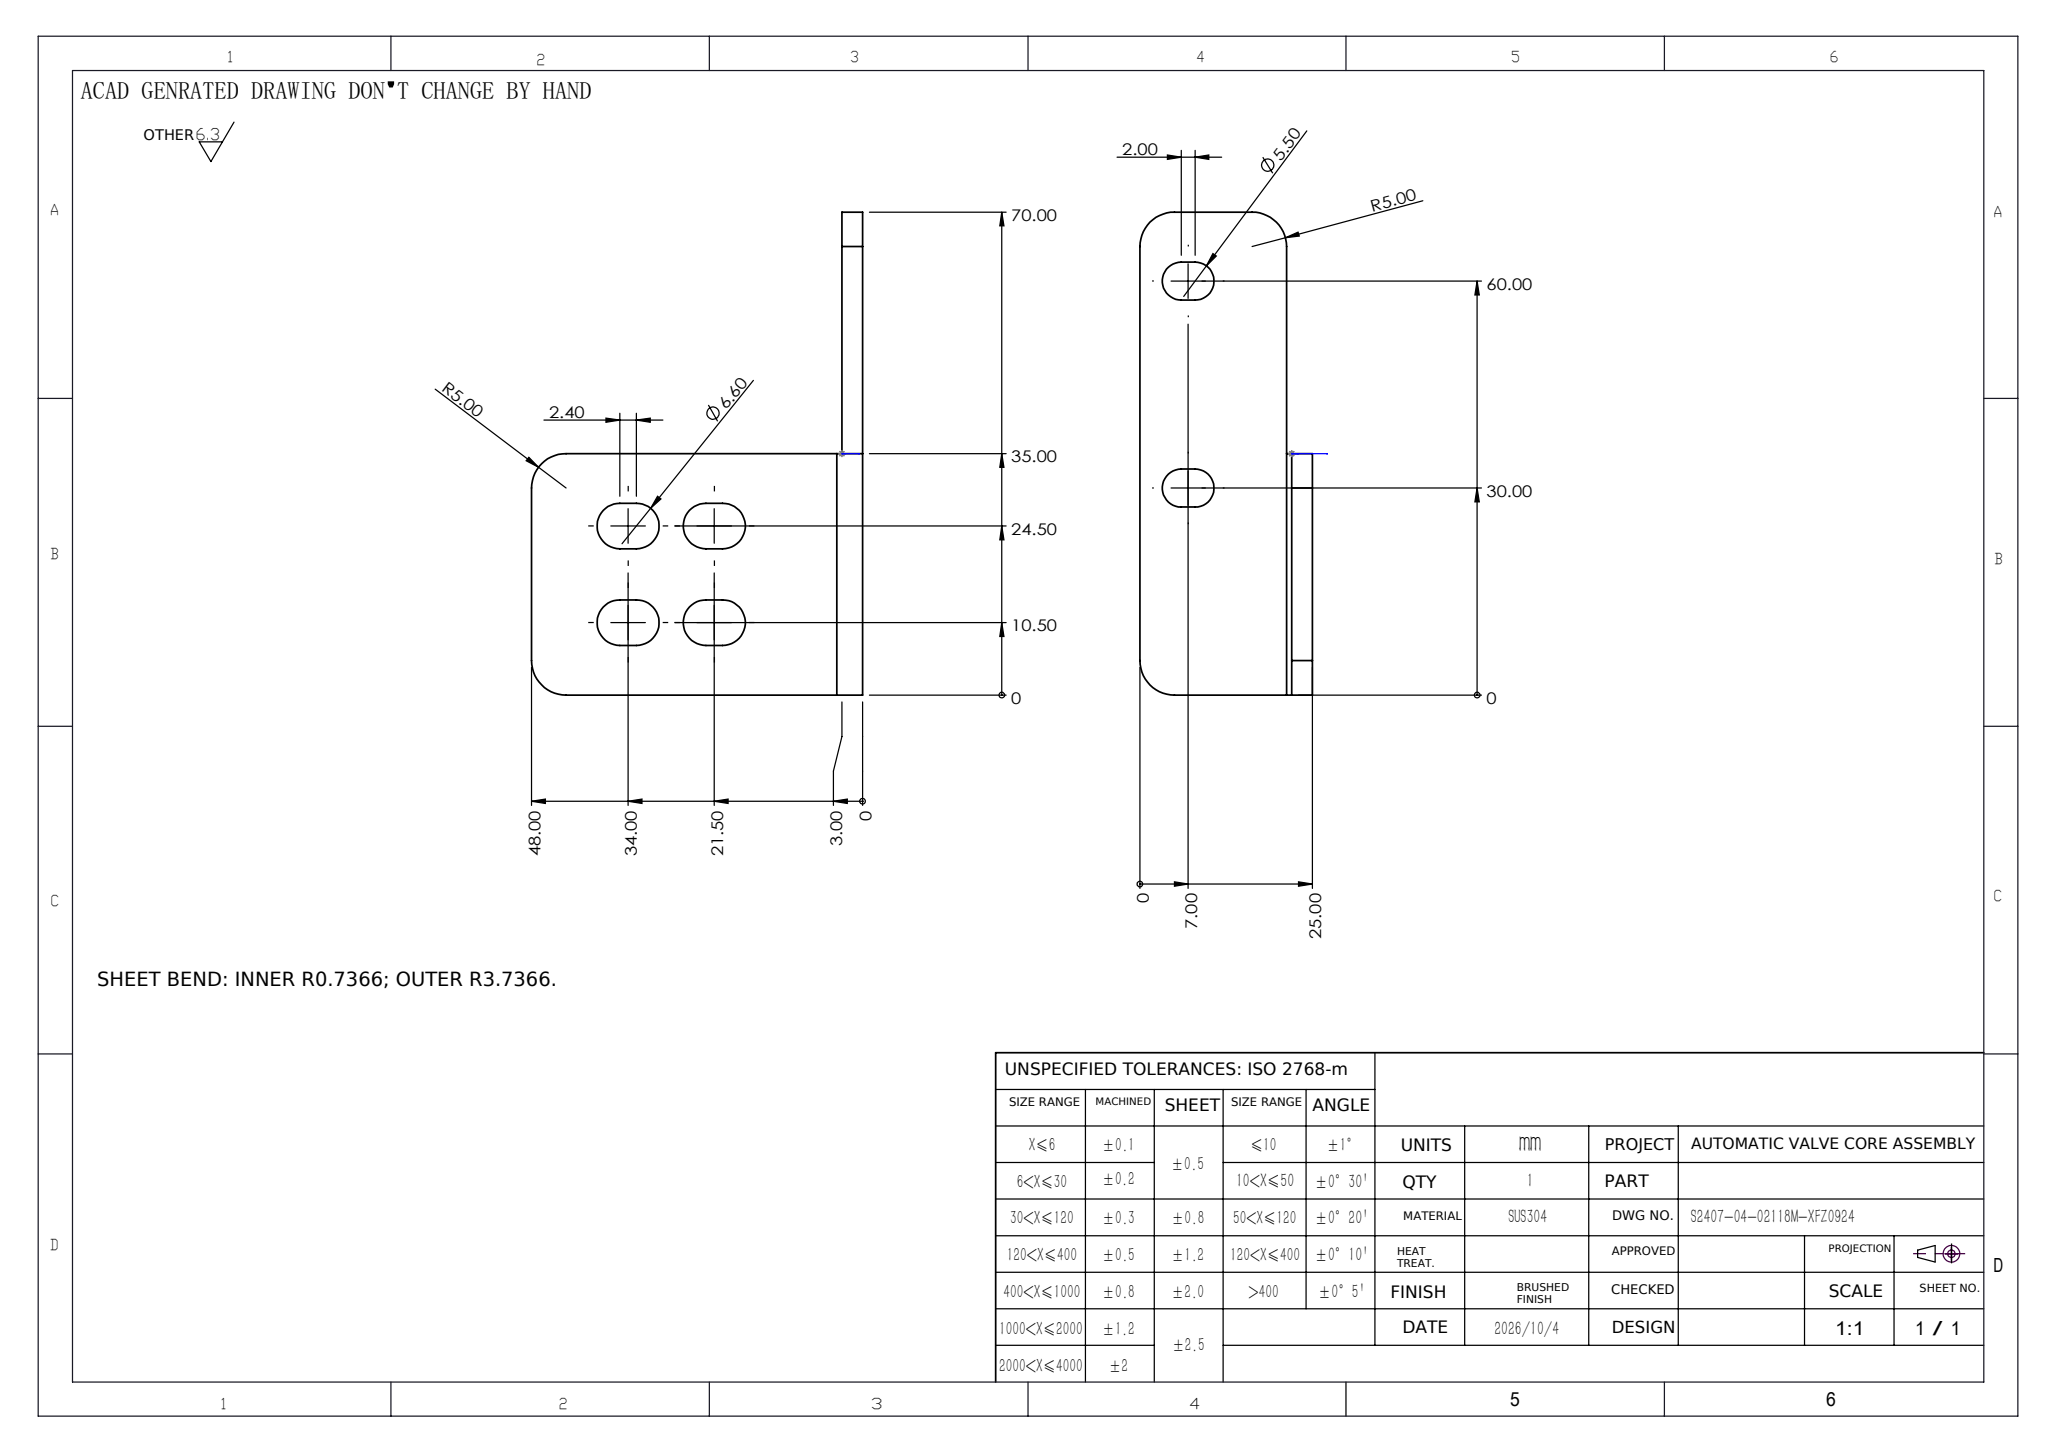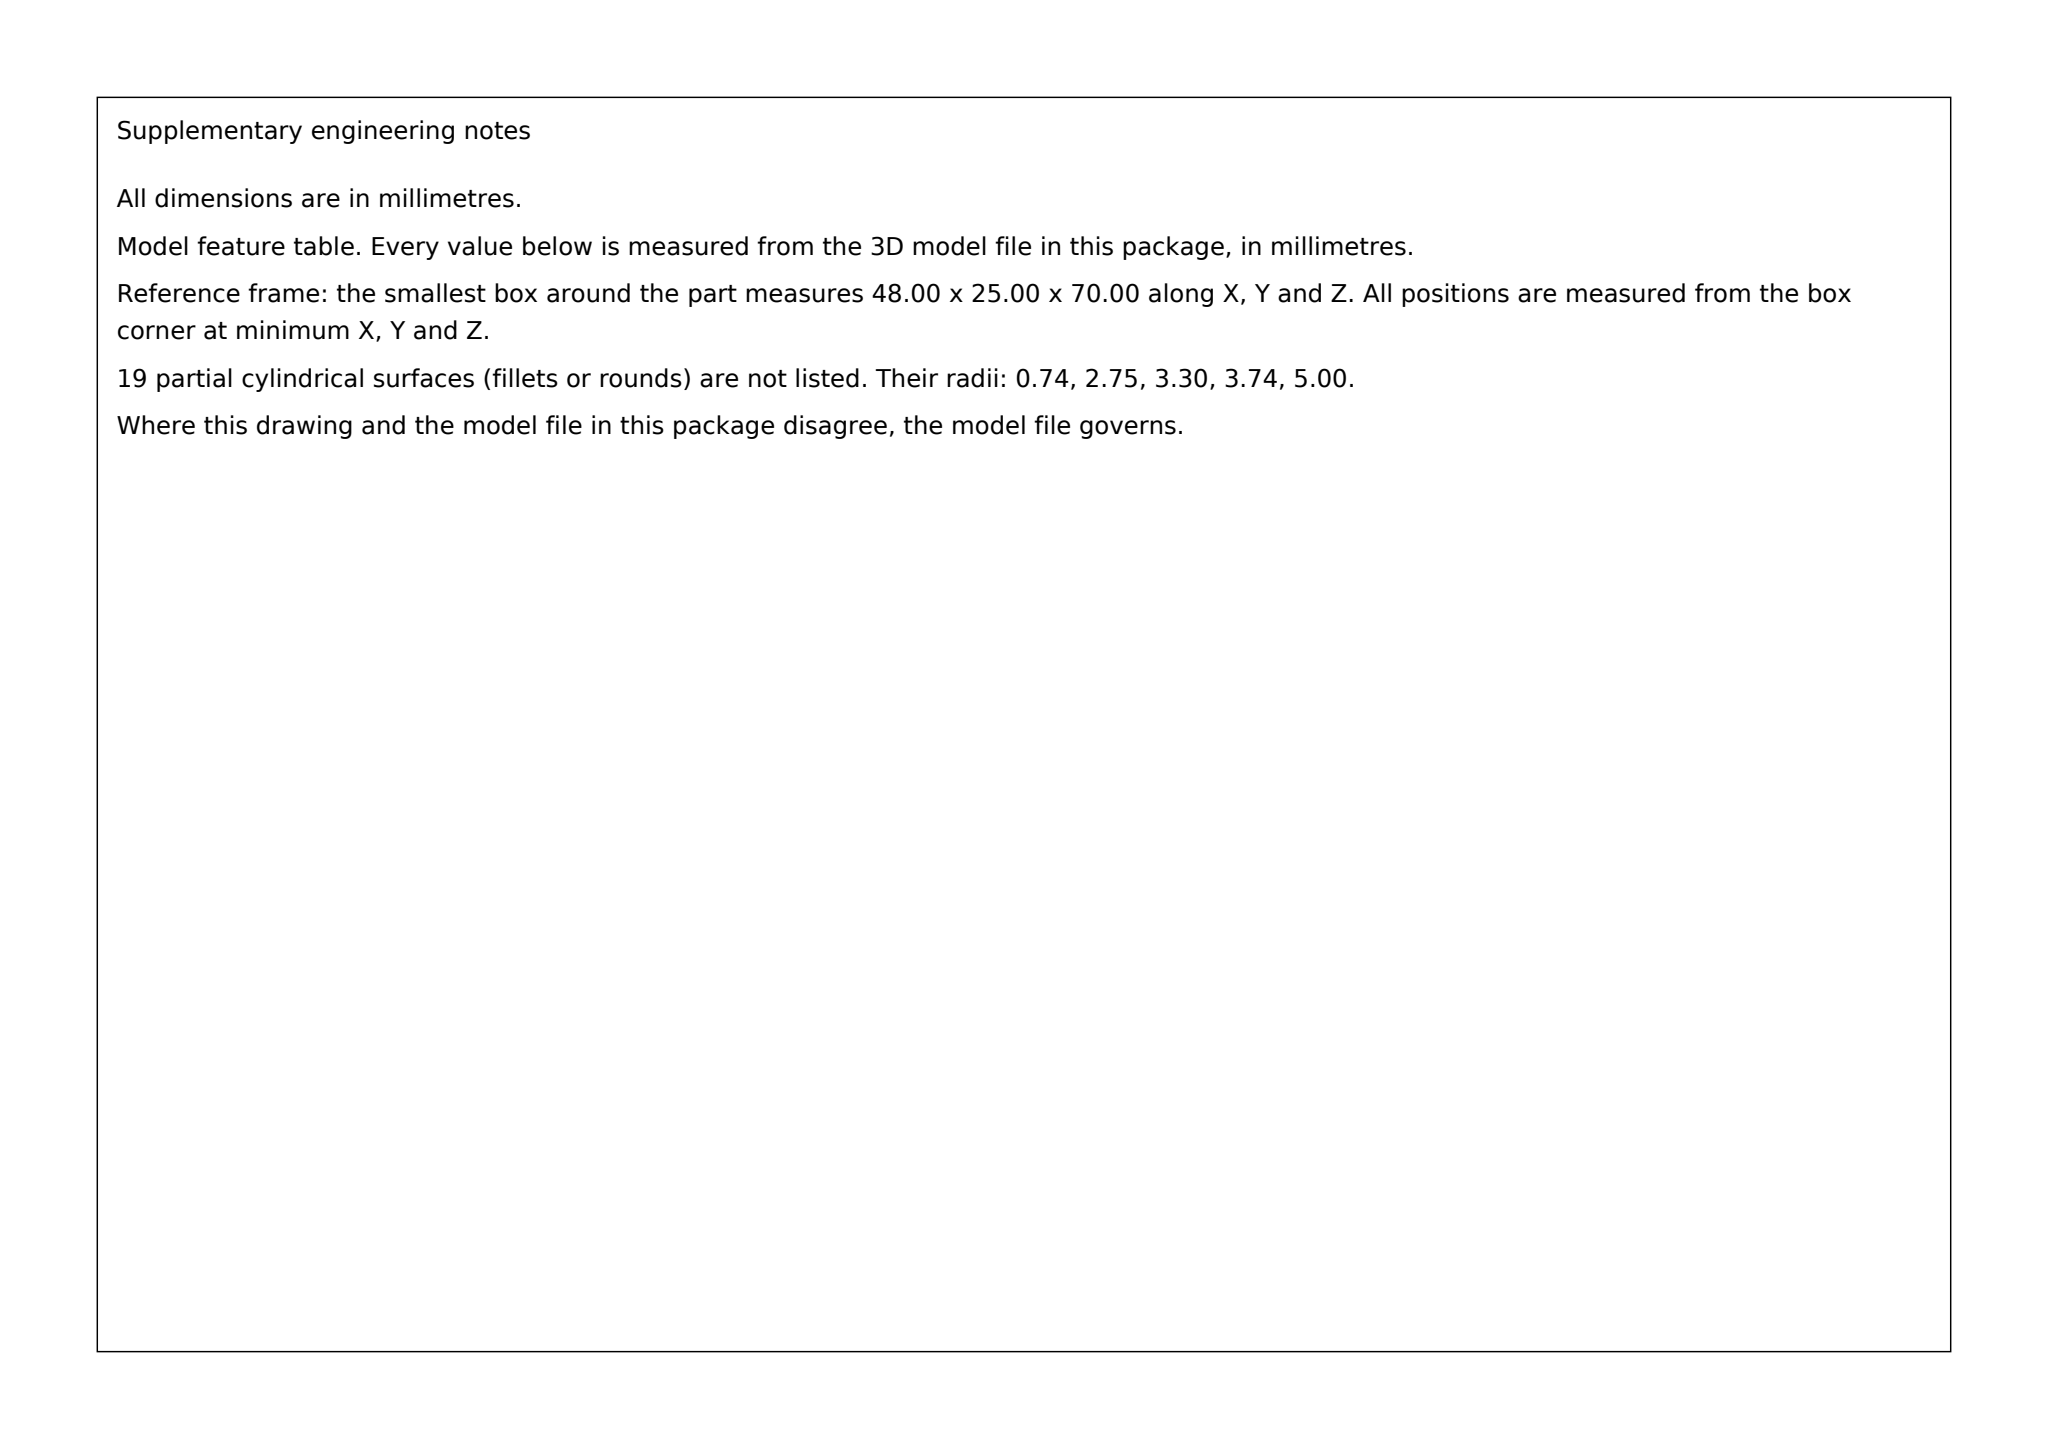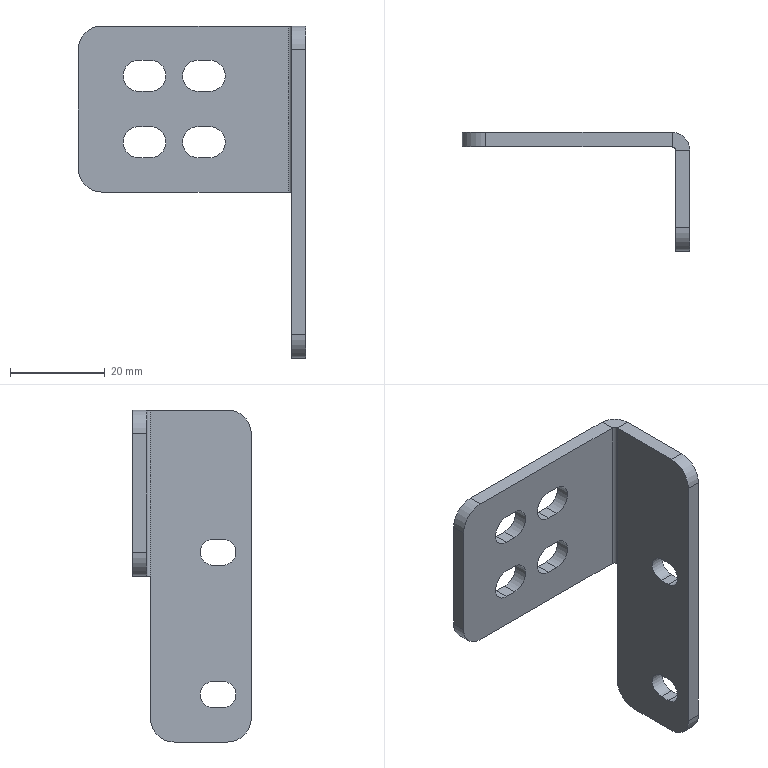Part | SolidWorks | mm | 1 solid | 43 faces | box 48 x 25 x 70 mm | volume 8592 mm3 | plane 24 | cylinder 19 | commonest cylinder face diameters 6.6 x8 10 x5 5.5 x4 1.473 x1 7.473 x1